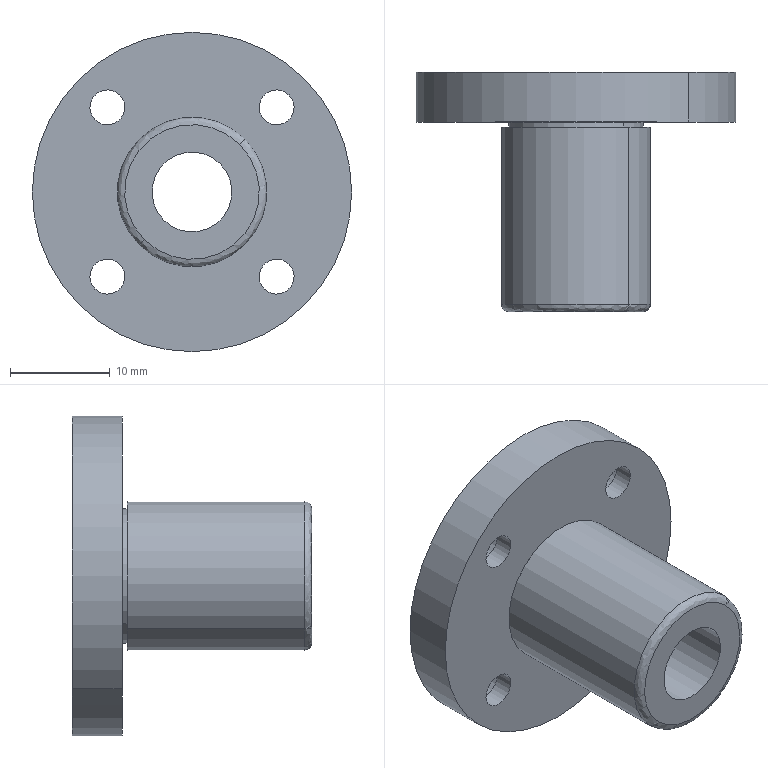Component | SolidWorks | LinearBearingLHFR8-1 | 1 solid | 34 faces | box 32 x 24 x 32 mm | volume 5726 mm3 | cylinder 24 | plane 7 | spline 3 | commonest cylinder face diameters 6 x8 3.5 x8 32 x2 8 x2 13.5 x2 15 x2
STEP:
#1=COLOUR_RGB('',0.7922,0.8196,0.9333);
#2=FILL_AREA_STYLE_COLOUR('',#1);
#3=FILL_AREA_STYLE('',(#2));
#4=SURFACE_STYLE_FILL_AREA(#3);
#5=SURFACE_SIDE_STYLE('',(#4));
#6=SURFACE_STYLE_USAGE(.BOTH.,#5);
#7=PRESENTATION_STYLE_ASSIGNMENT((#6));
#8=CARTESIAN_POINT('',(0.03812,2.123,-4.792));
#9=VERTEX_POINT('',#8);
#10=CARTESIAN_POINT('',(-0.3795,2.123,-5.209));
#11=VERTEX_POINT('',#10);
#12=CARTESIAN_POINT('',(-0.1707,2.123,-5.001));
#13=DIRECTION('',(0.,-1.,0.));
#14=DIRECTION('',(0.7071,0.,0.7071));
#15=AXIS2_PLACEMENT_3D('',#12,#13,#14);
#16=CIRCLE('',#15,0.2953);
#17=EDGE_CURVE('',#9,#11,#16,.T.);
#18=ORIENTED_EDGE('',*,*,#17,.T.);
#19=CARTESIAN_POINT('',(-0.3586,2.093,-5.188));
#20=VERTEX_POINT('',#19);
#21=CARTESIAN_POINT('',(-0.3586,2.123,-5.188));
#22=DIRECTION('',(-0.7071,0.,0.7071));
#23=DIRECTION('',(0.7071,0.,0.7071));
#24=AXIS2_PLACEMENT_3D('',#21,#22,#23);
#25=CIRCLE('',#24,0.02953);
#26=EDGE_CURVE('',#11,#20,#25,.T.);
#27=ORIENTED_EDGE('',*,*,#26,.T.);
#28=CARTESIAN_POINT('',(0.01724,2.093,-4.813));
#29=VERTEX_POINT('',#28);
#30=CARTESIAN_POINT('',(-0.1707,2.093,-5.001));
#31=DIRECTION('',(0.,-1.,0.));
#32=DIRECTION('',(0.7071,0.,0.7071));
#33=AXIS2_PLACEMENT_3D('',#30,#31,#32);
#34=CIRCLE('',#33,0.2657);
#35=EDGE_CURVE('',#29,#20,#34,.T.);
#36=ORIENTED_EDGE('',*,*,#35,.F.);
#37=CARTESIAN_POINT('',(0.01724,2.123,-4.813));
#38=DIRECTION('',(0.7071,0.,-0.7071));
#39=DIRECTION('',(-0.7071,0.,-0.7071));
#40=AXIS2_PLACEMENT_3D('',#37,#38,#39);
#41=CIRCLE('',#40,0.02953);
#42=EDGE_CURVE('',#9,#29,#41,.T.);
#43=ORIENTED_EDGE('',*,*,#42,.F.);
#44=EDGE_LOOP('',(#18,#27,#36,#43));
#45=FACE_OUTER_BOUND('',#44,.T.);
#46=CARTESIAN_POINT('',(-0.3795,2.123,-5.209));
#47=CARTESIAN_POINT('',(-0.7971,2.123,-4.792));
#48=CARTESIAN_POINT('',(-0.3795,2.123,-4.374));
#49=CARTESIAN_POINT('',(0.03812,2.123,-4.792));
#50=CARTESIAN_POINT('',(-0.3795,2.105,-5.209));
#51=CARTESIAN_POINT('',(-0.7971,2.105,-4.792));
#52=CARTESIAN_POINT('',(-0.3795,2.105,-4.374));
#53=CARTESIAN_POINT('',(0.03812,2.105,-4.792));
#54=CARTESIAN_POINT('',(-0.3708,2.093,-5.201));
#55=CARTESIAN_POINT('',(-0.7711,2.093,-4.8));
#56=CARTESIAN_POINT('',(-0.3708,2.093,-4.4));
#57=CARTESIAN_POINT('',(0.02947,2.093,-4.8));
#58=CARTESIAN_POINT('',(-0.3586,2.093,-5.188));
#59=CARTESIAN_POINT('',(-0.7344,2.093,-4.813));
#60=CARTESIAN_POINT('',(-0.3586,2.093,-4.437));
#61=CARTESIAN_POINT('',(0.01724,2.093,-4.813));
#62=(BOUNDED_SURFACE()B_SPLINE_SURFACE(3,3,((#46,#47,#48,#49),(#50,#51,#52,#53),(#54,#55,#56,#57),(#58,#59,#60,#61)),.UNSPECIFIED.,.F.,.F.,.T.)B_SPLINE_SURFACE_WITH_KNOTS((4,4),(4,4),(0.,1.),(0.,1.),.UNSPECIFIED.)GEOMETRIC_REPRESENTATION_ITEM()RATIONAL_B_SPLINE_SURFACE(((1.,0.3333,0.3333,1.),(0.8047,0.2682,0.2682,0.8047),(0.8047,0.2682,0.2682,0.8047),(1.,0.3333,0.3333,1.)))REPRESENTATION_ITEM('')SURFACE());
#63=ADVANCED_FACE('',(#45),#62,.T.);
#64=CARTESIAN_POINT('',(0.2747,2.841,-4.555));
#65=VERTEX_POINT('',#64);
#66=CARTESIAN_POINT('',(-0.6161,2.841,-5.446));
#67=VERTEX_POINT('',#66);
#68=CARTESIAN_POINT('',(-0.1707,2.841,-5.001));
#69=DIRECTION('',(0.,1.,0.));
#70=DIRECTION('',(0.7071,0.,0.7071));
#71=AXIS2_PLACEMENT_3D('',#68,#69,#70);
#72=CIRCLE('',#71,0.6299);
#73=EDGE_CURVE('',#65,#67,#72,.T.);
#74=ORIENTED_EDGE('',*,*,#73,.T.);
#75=CARTESIAN_POINT('',(-0.6161,3.038,-5.446));
#76=VERTEX_POINT('',#75);
#77=CARTESIAN_POINT('',(-0.6161,3.038,-5.446));
#78=DIRECTION('',(0.,1.,0.));
#79=VECTOR('',#78,39.37);
#80=LINE('',#77,#79);
#81=EDGE_CURVE('',#67,#76,#80,.T.);
#82=ORIENTED_EDGE('',*,*,#81,.T.);
#83=CARTESIAN_POINT('',(0.2747,3.038,-4.555));
#84=VERTEX_POINT('',#83);
#85=CARTESIAN_POINT('',(-0.1707,3.038,-5.001));
#86=DIRECTION('',(0.,-1.,0.));
#87=DIRECTION('',(0.7071,0.,0.7071));
#88=AXIS2_PLACEMENT_3D('',#85,#86,#87);
#89=CIRCLE('',#88,0.6299);
#90=EDGE_CURVE('',#76,#84,#89,.T.);
#91=ORIENTED_EDGE('',*,*,#90,.T.);
#92=CARTESIAN_POINT('',(0.2747,3.038,-4.555));
#93=DIRECTION('',(0.,1.,0.));
#94=VECTOR('',#93,39.37);
#95=LINE('',#92,#94);
#96=EDGE_CURVE('',#65,#84,#95,.T.);
#97=ORIENTED_EDGE('',*,*,#96,.F.);
#98=EDGE_LOOP('',(#74,#82,#91,#97));
#99=FACE_OUTER_BOUND('',#98,.T.);
#100=CARTESIAN_POINT('',(-0.1707,3.038,-5.001));
#101=DIRECTION('',(0.,1.,0.));
#102=DIRECTION('',(0.7071,0.,0.7071));
#103=AXIS2_PLACEMENT_3D('',#100,#101,#102);
#104=CYLINDRICAL_SURFACE('',#103,0.6299);
#105=ADVANCED_FACE('',(#99),#104,.T.);
#106=CARTESIAN_POINT('',(-0.05932,2.093,-4.889));
#107=VERTEX_POINT('',#106);
#108=CARTESIAN_POINT('',(-0.282,2.093,-5.112));
#109=VERTEX_POINT('',#108);
#110=CARTESIAN_POINT('',(-0.1707,2.093,-5.001));
#111=DIRECTION('',(0.,-1.,0.));
#112=DIRECTION('',(0.7071,0.,0.7071));
#113=AXIS2_PLACEMENT_3D('',#110,#111,#112);
#114=CIRCLE('',#113,0.1575);
#115=EDGE_CURVE('',#107,#109,#114,.T.);
#116=ORIENTED_EDGE('',*,*,#115,.T.);
#117=CARTESIAN_POINT('',(-0.282,3.038,-5.112));
#118=VERTEX_POINT('',#117);
#119=CARTESIAN_POINT('',(-0.282,2.093,-5.112));
#120=DIRECTION('',(0.,1.,0.));
#121=VECTOR('',#120,39.37);
#122=LINE('',#119,#121);
#123=EDGE_CURVE('',#109,#118,#122,.T.);
#124=ORIENTED_EDGE('',*,*,#123,.T.);
#125=CARTESIAN_POINT('',(-0.05932,3.038,-4.889));
#126=VERTEX_POINT('',#125);
#127=CARTESIAN_POINT('',(-0.1707,3.038,-5.001));
#128=DIRECTION('',(0.,-1.,0.));
#129=DIRECTION('',(0.7071,0.,0.7071));
#130=AXIS2_PLACEMENT_3D('',#127,#128,#129);
#131=CIRCLE('',#130,0.1575);
#132=EDGE_CURVE('',#126,#118,#131,.T.);
#133=ORIENTED_EDGE('',*,*,#132,.F.);
#134=CARTESIAN_POINT('',(-0.05932,2.093,-4.889));
#135=DIRECTION('',(0.,1.,0.));
#136=VECTOR('',#135,39.37);
#137=LINE('',#134,#136);
#138=EDGE_CURVE('',#107,#126,#137,.T.);
#139=ORIENTED_EDGE('',*,*,#138,.F.);
#140=EDGE_LOOP('',(#116,#124,#133,#139));
#141=FACE_OUTER_BOUND('',#140,.T.);
#142=CARTESIAN_POINT('',(-0.1707,2.093,-5.001));
#143=DIRECTION('',(0.,1.,0.));
#144=DIRECTION('',(0.7071,0.,0.7071));
#145=AXIS2_PLACEMENT_3D('',#142,#143,#144);
#146=CYLINDRICAL_SURFACE('',#145,0.1575);
#147=ADVANCED_FACE('',(#141),#146,.F.);
#148=CARTESIAN_POINT('',(0.2469,2.916,-5.251));
#149=VERTEX_POINT('',#148);
#150=CARTESIAN_POINT('',(0.07987,2.916,-5.418));
#151=VERTEX_POINT('',#150);
#152=CARTESIAN_POINT('',(0.1634,2.916,-5.335));
#153=DIRECTION('',(0.,-1.,0.));
#154=DIRECTION('',(0.7071,0.,0.7071));
#155=AXIS2_PLACEMENT_3D('',#152,#153,#154);
#156=CIRCLE('',#155,0.1181);
#157=EDGE_CURVE('',#149,#151,#156,.T.);
#158=ORIENTED_EDGE('',*,*,#157,.T.);
#159=CARTESIAN_POINT('',(0.07987,3.038,-5.418));
#160=VERTEX_POINT('',#159);
#161=CARTESIAN_POINT('',(0.07987,2.916,-5.418));
#162=DIRECTION('',(0.,1.,0.));
#163=VECTOR('',#162,39.37);
#164=LINE('',#161,#163);
#165=EDGE_CURVE('',#151,#160,#164,.T.);
#166=ORIENTED_EDGE('',*,*,#165,.T.);
#167=CARTESIAN_POINT('',(0.2469,3.038,-5.251));
#168=VERTEX_POINT('',#167);
#169=CARTESIAN_POINT('',(0.1634,3.038,-5.335));
#170=DIRECTION('',(0.,-1.,0.));
#171=DIRECTION('',(0.7071,0.,0.7071));
#172=AXIS2_PLACEMENT_3D('',#169,#170,#171);
#173=CIRCLE('',#172,0.1181);
#174=EDGE_CURVE('',#168,#160,#173,.T.);
#175=ORIENTED_EDGE('',*,*,#174,.F.);
#176=CARTESIAN_POINT('',(0.2469,2.916,-5.251));
#177=DIRECTION('',(0.,1.,0.));
#178=VECTOR('',#177,39.37);
#179=LINE('',#176,#178);
#180=EDGE_CURVE('',#149,#168,#179,.T.);
#181=ORIENTED_EDGE('',*,*,#180,.F.);
#182=EDGE_LOOP('',(#158,#166,#175,#181));
#183=FACE_OUTER_BOUND('',#182,.T.);
#184=CARTESIAN_POINT('',(0.1634,2.916,-5.335));
#185=DIRECTION('',(0.,1.,0.));
#186=DIRECTION('',(0.7071,0.,0.7071));
#187=AXIS2_PLACEMENT_3D('',#184,#185,#186);
#188=CYLINDRICAL_SURFACE('',#187,0.1181);
#189=ADVANCED_FACE('',(#183),#188,.F.);
#190=CARTESIAN_POINT('',(-0.4212,2.916,-5.251));
#191=VERTEX_POINT('',#190);
#192=CARTESIAN_POINT('',(-0.5883,2.916,-5.418));
#193=VERTEX_POINT('',#192);
#194=CARTESIAN_POINT('',(-0.5047,2.916,-5.335));
#195=DIRECTION('',(0.,-1.,0.));
#196=DIRECTION('',(0.7071,0.,0.7071));
#197=AXIS2_PLACEMENT_3D('',#194,#195,#196);
#198=CIRCLE('',#197,0.1181);
#199=EDGE_CURVE('',#191,#193,#198,.T.);
#200=ORIENTED_EDGE('',*,*,#199,.T.);
#201=CARTESIAN_POINT('',(-0.5883,3.038,-5.418));
#202=VERTEX_POINT('',#201);
#203=CARTESIAN_POINT('',(-0.5883,2.916,-5.418));
#204=DIRECTION('',(0.,1.,0.));
#205=VECTOR('',#204,39.37);
#206=LINE('',#203,#205);
#207=EDGE_CURVE('',#193,#202,#206,.T.);
#208=ORIENTED_EDGE('',*,*,#207,.T.);
#209=CARTESIAN_POINT('',(-0.4212,3.038,-5.251));
#210=VERTEX_POINT('',#209);
#211=CARTESIAN_POINT('',(-0.5047,3.038,-5.335));
#212=DIRECTION('',(0.,-1.,0.));
#213=DIRECTION('',(0.7071,0.,0.7071));
#214=AXIS2_PLACEMENT_3D('',#211,#212,#213);
#215=CIRCLE('',#214,0.1181);
#216=EDGE_CURVE('',#210,#202,#215,.T.);
#217=ORIENTED_EDGE('',*,*,#216,.F.);
#218=CARTESIAN_POINT('',(-0.4212,2.916,-5.251));
#219=DIRECTION('',(0.,1.,0.));
#220=VECTOR('',#219,39.37);
#221=LINE('',#218,#220);
#222=EDGE_CURVE('',#191,#210,#221,.T.);
#223=ORIENTED_EDGE('',*,*,#222,.F.);
#224=EDGE_LOOP('',(#200,#208,#217,#223));
#225=FACE_OUTER_BOUND('',#224,.T.);
#226=CARTESIAN_POINT('',(-0.5047,2.916,-5.335));
#227=DIRECTION('',(0.,1.,0.));
#228=DIRECTION('',(0.7071,0.,0.7071));
#229=AXIS2_PLACEMENT_3D('',#226,#227,#228);
#230=CYLINDRICAL_SURFACE('',#229,0.1181);
#231=ADVANCED_FACE('',(#225),#230,.F.);
#232=CARTESIAN_POINT('',(-0.4212,2.916,-4.583));
#233=VERTEX_POINT('',#232);
#234=CARTESIAN_POINT('',(-0.5883,2.916,-4.75));
#235=VERTEX_POINT('',#234);
#236=CARTESIAN_POINT('',(-0.5047,2.916,-4.667));
#237=DIRECTION('',(0.,-1.,0.));
#238=DIRECTION('',(0.7071,0.,0.7071));
#239=AXIS2_PLACEMENT_3D('',#236,#237,#238);
#240=CIRCLE('',#239,0.1181);
#241=EDGE_CURVE('',#233,#235,#240,.T.);
#242=ORIENTED_EDGE('',*,*,#241,.T.);
#243=CARTESIAN_POINT('',(-0.5883,3.038,-4.75));
#244=VERTEX_POINT('',#243);
#245=CARTESIAN_POINT('',(-0.5883,2.916,-4.75));
#246=DIRECTION('',(0.,1.,0.));
#247=VECTOR('',#246,39.37);
#248=LINE('',#245,#247);
#249=EDGE_CURVE('',#235,#244,#248,.T.);
#250=ORIENTED_EDGE('',*,*,#249,.T.);
#251=CARTESIAN_POINT('',(-0.4212,3.038,-4.583));
#252=VERTEX_POINT('',#251);
#253=CARTESIAN_POINT('',(-0.5047,3.038,-4.667));
#254=DIRECTION('',(0.,-1.,0.));
#255=DIRECTION('',(0.7071,0.,0.7071));
#256=AXIS2_PLACEMENT_3D('',#253,#254,#255);
#257=CIRCLE('',#256,0.1181);
#258=EDGE_CURVE('',#252,#244,#257,.T.);
#259=ORIENTED_EDGE('',*,*,#258,.F.);
#260=CARTESIAN_POINT('',(-0.4212,2.916,-4.583));
#261=DIRECTION('',(0.,1.,0.));
#262=VECTOR('',#261,39.37);
#263=LINE('',#260,#262);
#264=EDGE_CURVE('',#233,#252,#263,.T.);
#265=ORIENTED_EDGE('',*,*,#264,.F.);
#266=EDGE_LOOP('',(#242,#250,#259,#265));
#267=FACE_OUTER_BOUND('',#266,.T.);
#268=CARTESIAN_POINT('',(-0.5047,2.916,-4.667));
#269=DIRECTION('',(0.,1.,0.));
#270=DIRECTION('',(0.7071,0.,0.7071));
#271=AXIS2_PLACEMENT_3D('',#268,#269,#270);
#272=CYLINDRICAL_SURFACE('',#271,0.1181);
#273=ADVANCED_FACE('',(#267),#272,.F.);
#274=CARTESIAN_POINT('',(0.2469,2.916,-4.583));
#275=VERTEX_POINT('',#274);
#276=CARTESIAN_POINT('',(0.07987,2.916,-4.75));
#277=VERTEX_POINT('',#276);
#278=CARTESIAN_POINT('',(0.1634,2.916,-4.667));
#279=DIRECTION('',(0.,-1.,0.));
#280=DIRECTION('',(0.7071,0.,0.7071));
#281=AXIS2_PLACEMENT_3D('',#278,#279,#280);
#282=CIRCLE('',#281,0.1181);
#283=EDGE_CURVE('',#275,#277,#282,.T.);
#284=ORIENTED_EDGE('',*,*,#283,.T.);
#285=CARTESIAN_POINT('',(0.07987,3.038,-4.75));
#286=VERTEX_POINT('',#285);
#287=CARTESIAN_POINT('',(0.07987,2.916,-4.75));
#288=DIRECTION('',(0.,1.,0.));
#289=VECTOR('',#288,39.37);
#290=LINE('',#287,#289);
#291=EDGE_CURVE('',#277,#286,#290,.T.);
#292=ORIENTED_EDGE('',*,*,#291,.T.);
#293=CARTESIAN_POINT('',(0.2469,3.038,-4.583));
#294=VERTEX_POINT('',#293);
#295=CARTESIAN_POINT('',(0.1634,3.038,-4.667));
#296=DIRECTION('',(0.,-1.,0.));
#297=DIRECTION('',(0.7071,0.,0.7071));
#298=AXIS2_PLACEMENT_3D('',#295,#296,#297);
#299=CIRCLE('',#298,0.1181);
#300=EDGE_CURVE('',#294,#286,#299,.T.);
#301=ORIENTED_EDGE('',*,*,#300,.F.);
#302=CARTESIAN_POINT('',(0.2469,2.916,-4.583));
#303=DIRECTION('',(0.,1.,0.));
#304=VECTOR('',#303,39.37);
#305=LINE('',#302,#304);
#306=EDGE_CURVE('',#275,#294,#305,.T.);
#307=ORIENTED_EDGE('',*,*,#306,.F.);
#308=EDGE_LOOP('',(#284,#292,#301,#307));
#309=FACE_OUTER_BOUND('',#308,.T.);
#310=CARTESIAN_POINT('',(0.1634,2.916,-4.667));
#311=DIRECTION('',(0.,1.,0.));
#312=DIRECTION('',(0.7071,0.,0.7071));
#313=AXIS2_PLACEMENT_3D('',#310,#311,#312);
#314=CYLINDRICAL_SURFACE('',#313,0.1181);
#315=ADVANCED_FACE('',(#309),#314,.F.);
#316=CARTESIAN_POINT('',(0.01724,2.822,-4.813));
#317=VERTEX_POINT('',#316);
#318=CARTESIAN_POINT('',(-0.3586,2.822,-5.188));
#319=VERTEX_POINT('',#318);
#320=CARTESIAN_POINT('',(-0.1707,2.822,-5.001));
#321=DIRECTION('',(0.,1.,0.));
#322=DIRECTION('',(0.7071,0.,0.7071));
#323=AXIS2_PLACEMENT_3D('',#320,#321,#322);
#324=CIRCLE('',#323,0.2657);
#325=EDGE_CURVE('',#317,#319,#324,.T.);
#326=ORIENTED_EDGE('',*,*,#325,.T.);
#327=CARTESIAN_POINT('',(-0.3586,2.841,-5.188));
#328=VERTEX_POINT('',#327);
#329=CARTESIAN_POINT('',(-0.3586,2.841,-5.188));
#330=DIRECTION('',(0.,1.,0.));
#331=VECTOR('',#330,39.37);
#332=LINE('',#329,#331);
#333=EDGE_CURVE('',#319,#328,#332,.T.);
#334=ORIENTED_EDGE('',*,*,#333,.T.);
#335=CARTESIAN_POINT('',(0.01724,2.841,-4.813));
#336=VERTEX_POINT('',#335);
#337=CARTESIAN_POINT('',(-0.1707,2.841,-5.001));
#338=DIRECTION('',(0.,1.,0.));
#339=DIRECTION('',(0.7071,0.,0.7071));
#340=AXIS2_PLACEMENT_3D('',#337,#338,#339);
#341=CIRCLE('',#340,0.2657);
#342=EDGE_CURVE('',#336,#328,#341,.T.);
#343=ORIENTED_EDGE('',*,*,#342,.F.);
#344=CARTESIAN_POINT('',(0.01724,2.841,-4.813));
#345=DIRECTION('',(0.,1.,0.));
#346=VECTOR('',#345,39.37);
#347=LINE('',#344,#346);
#348=EDGE_CURVE('',#317,#336,#347,.T.);
#349=ORIENTED_EDGE('',*,*,#348,.F.);
#350=EDGE_LOOP('',(#326,#334,#343,#349));
#351=FACE_OUTER_BOUND('',#350,.T.);
#352=CARTESIAN_POINT('',(-0.1707,2.841,-5.001));
#353=DIRECTION('',(0.,1.,0.));
#354=DIRECTION('',(0.7071,0.,0.7071));
#355=AXIS2_PLACEMENT_3D('',#352,#353,#354);
#356=CYLINDRICAL_SURFACE('',#355,0.2657);
#357=ADVANCED_FACE('',(#351),#356,.T.);
#358=CARTESIAN_POINT('',(0.1147,2.841,-5.383));
#359=VERTEX_POINT('',#358);
#360=CARTESIAN_POINT('',(0.2121,2.841,-5.286));
#361=VERTEX_POINT('',#360);
#362=CARTESIAN_POINT('',(0.1634,2.841,-5.335));
#363=DIRECTION('',(0.,1.,0.));
#364=DIRECTION('',(0.7071,0.,0.7071));
#365=AXIS2_PLACEMENT_3D('',#362,#363,#364);
#366=CIRCLE('',#365,0.0689);
#367=EDGE_CURVE('',#359,#361,#366,.T.);
#368=ORIENTED_EDGE('',*,*,#367,.F.);
#369=CARTESIAN_POINT('',(0.1147,2.916,-5.383));
#370=VERTEX_POINT('',#369);
#371=CARTESIAN_POINT('',(0.1147,2.841,-5.383));
#372=DIRECTION('',(0.,1.,0.));
#373=VECTOR('',#372,39.37);
#374=LINE('',#371,#373);
#375=EDGE_CURVE('',#359,#370,#374,.T.);
#376=ORIENTED_EDGE('',*,*,#375,.T.);
#377=CARTESIAN_POINT('',(0.2121,2.916,-5.286));
#378=VERTEX_POINT('',#377);
#379=CARTESIAN_POINT('',(0.1634,2.916,-5.335));
#380=DIRECTION('',(0.,1.,0.));
#381=DIRECTION('',(0.7071,0.,0.7071));
#382=AXIS2_PLACEMENT_3D('',#379,#380,#381);
#383=CIRCLE('',#382,0.0689);
#384=EDGE_CURVE('',#370,#378,#383,.T.);
#385=ORIENTED_EDGE('',*,*,#384,.T.);
#386=CARTESIAN_POINT('',(0.2121,2.841,-5.286));
#387=DIRECTION('',(0.,1.,0.));
#388=VECTOR('',#387,39.37);
#389=LINE('',#386,#388);
#390=EDGE_CURVE('',#361,#378,#389,.T.);
#391=ORIENTED_EDGE('',*,*,#390,.F.);
#392=EDGE_LOOP('',(#368,#376,#385,#391));
#393=FACE_OUTER_BOUND('',#392,.T.);
#394=CARTESIAN_POINT('',(0.1634,2.841,-5.335));
#395=DIRECTION('',(0.,1.,0.));
#396=DIRECTION('',(0.7071,0.,0.7071));
#397=AXIS2_PLACEMENT_3D('',#394,#395,#396);
#398=CYLINDRICAL_SURFACE('',#397,0.0689);
#399=ADVANCED_FACE('',(#393),#398,.F.);
#400=CARTESIAN_POINT('',(-0.5535,2.841,-5.383));
#401=VERTEX_POINT('',#400);
#402=CARTESIAN_POINT('',(-0.456,2.841,-5.286));
#403=VERTEX_POINT('',#402);
#404=CARTESIAN_POINT('',(-0.5047,2.841,-5.335));
#405=DIRECTION('',(0.,1.,0.));
#406=DIRECTION('',(0.7071,0.,0.7071));
#407=AXIS2_PLACEMENT_3D('',#404,#405,#406);
#408=CIRCLE('',#407,0.0689);
#409=EDGE_CURVE('',#401,#403,#408,.T.);
#410=ORIENTED_EDGE('',*,*,#409,.F.);
#411=CARTESIAN_POINT('',(-0.5535,2.916,-5.383));
#412=VERTEX_POINT('',#411);
#413=CARTESIAN_POINT('',(-0.5535,2.841,-5.383));
#414=DIRECTION('',(0.,1.,0.));
#415=VECTOR('',#414,39.37);
#416=LINE('',#413,#415);
#417=EDGE_CURVE('',#401,#412,#416,.T.);
#418=ORIENTED_EDGE('',*,*,#417,.T.);
#419=CARTESIAN_POINT('',(-0.456,2.916,-5.286));
#420=VERTEX_POINT('',#419);
#421=CARTESIAN_POINT('',(-0.5047,2.916,-5.335));
#422=DIRECTION('',(0.,1.,0.));
#423=DIRECTION('',(0.7071,0.,0.7071));
#424=AXIS2_PLACEMENT_3D('',#421,#422,#423);
#425=CIRCLE('',#424,0.0689);
#426=EDGE_CURVE('',#412,#420,#425,.T.);
#427=ORIENTED_EDGE('',*,*,#426,.T.);
#428=CARTESIAN_POINT('',(-0.456,2.841,-5.286));
#429=DIRECTION('',(0.,1.,0.));
#430=VECTOR('',#429,39.37);
#431=LINE('',#428,#430);
#432=EDGE_CURVE('',#403,#420,#431,.T.);
#433=ORIENTED_EDGE('',*,*,#432,.F.);
#434=EDGE_LOOP('',(#410,#418,#427,#433));
#435=FACE_OUTER_BOUND('',#434,.T.);
#436=CARTESIAN_POINT('',(-0.5047,2.841,-5.335));
#437=DIRECTION('',(0.,1.,0.));
#438=DIRECTION('',(0.7071,0.,0.7071));
#439=AXIS2_PLACEMENT_3D('',#436,#437,#438);
#440=CYLINDRICAL_SURFACE('',#439,0.0689);
#441=ADVANCED_FACE('',(#435),#440,.F.);
#442=CARTESIAN_POINT('',(-0.5535,2.841,-4.715));
#443=VERTEX_POINT('',#442);
#444=CARTESIAN_POINT('',(-0.456,2.841,-4.618));
#445=VERTEX_POINT('',#444);
#446=CARTESIAN_POINT('',(-0.5047,2.841,-4.667));
#447=DIRECTION('',(0.,1.,0.));
#448=DIRECTION('',(0.7071,0.,0.7071));
#449=AXIS2_PLACEMENT_3D('',#446,#447,#448);
#450=CIRCLE('',#449,0.0689);
#451=EDGE_CURVE('',#443,#445,#450,.T.);
#452=ORIENTED_EDGE('',*,*,#451,.F.);
#453=CARTESIAN_POINT('',(-0.5535,2.916,-4.715));
#454=VERTEX_POINT('',#453);
#455=CARTESIAN_POINT('',(-0.5535,2.841,-4.715));
#456=DIRECTION('',(0.,1.,0.));
#457=VECTOR('',#456,39.37);
#458=LINE('',#455,#457);
#459=EDGE_CURVE('',#443,#454,#458,.T.);
#460=ORIENTED_EDGE('',*,*,#459,.T.);
#461=CARTESIAN_POINT('',(-0.456,2.916,-4.618));
#462=VERTEX_POINT('',#461);
#463=CARTESIAN_POINT('',(-0.5047,2.916,-4.667));
#464=DIRECTION('',(0.,1.,0.));
#465=DIRECTION('',(0.7071,0.,0.7071));
#466=AXIS2_PLACEMENT_3D('',#463,#464,#465);
#467=CIRCLE('',#466,0.0689);
#468=EDGE_CURVE('',#454,#462,#467,.T.);
#469=ORIENTED_EDGE('',*,*,#468,.T.);
#470=CARTESIAN_POINT('',(-0.456,2.841,-4.618));
#471=DIRECTION('',(0.,1.,0.));
#472=VECTOR('',#471,39.37);
#473=LINE('',#470,#472);
#474=EDGE_CURVE('',#445,#462,#473,.T.);
#475=ORIENTED_EDGE('',*,*,#474,.F.);
#476=EDGE_LOOP('',(#452,#460,#469,#475));
#477=FACE_OUTER_BOUND('',#476,.T.);
#478=CARTESIAN_POINT('',(-0.5047,2.841,-4.667));
#479=DIRECTION('',(0.,1.,0.));
#480=DIRECTION('',(0.7071,0.,0.7071));
#481=AXIS2_PLACEMENT_3D('',#478,#479,#480);
#482=CYLINDRICAL_SURFACE('',#481,0.0689);
#483=ADVANCED_FACE('',(#477),#482,.F.);
#484=CARTESIAN_POINT('',(0.1147,2.841,-4.715));
#485=VERTEX_POINT('',#484);
#486=CARTESIAN_POINT('',(0.2121,2.841,-4.618));
#487=VERTEX_POINT('',#486);
#488=CARTESIAN_POINT('',(0.1634,2.841,-4.667));
#489=DIRECTION('',(0.,1.,0.));
#490=DIRECTION('',(0.7071,0.,0.7071));
#491=AXIS2_PLACEMENT_3D('',#488,#489,#490);
#492=CIRCLE('',#491,0.0689);
#493=EDGE_CURVE('',#485,#487,#492,.T.);
#494=ORIENTED_EDGE('',*,*,#493,.F.);
#495=CARTESIAN_POINT('',(0.1147,2.916,-4.715));
#496=VERTEX_POINT('',#495);
#497=CARTESIAN_POINT('',(0.1147,2.841,-4.715));
#498=DIRECTION('',(0.,1.,0.));
#499=VECTOR('',#498,39.37);
#500=LINE('',#497,#499);
#501=EDGE_CURVE('',#485,#496,#500,.T.);
#502=ORIENTED_EDGE('',*,*,#501,.T.);
#503=CARTESIAN_POINT('',(0.2121,2.916,-4.618));
#504=VERTEX_POINT('',#503);
#505=CARTESIAN_POINT('',(0.1634,2.916,-4.667));
#506=DIRECTION('',(0.,1.,0.));
#507=DIRECTION('',(0.7071,0.,0.7071));
#508=AXIS2_PLACEMENT_3D('',#505,#506,#507);
#509=CIRCLE('',#508,0.0689);
#510=EDGE_CURVE('',#496,#504,#509,.T.);
#511=ORIENTED_EDGE('',*,*,#510,.T.);
#512=CARTESIAN_POINT('',(0.2121,2.841,-4.618));
#513=DIRECTION('',(0.,1.,0.));
#514=VECTOR('',#513,39.37);
#515=LINE('',#512,#514);
#516=EDGE_CURVE('',#487,#504,#515,.T.);
#517=ORIENTED_EDGE('',*,*,#516,.F.);
#518=EDGE_LOOP('',(#494,#502,#511,#517));
#519=FACE_OUTER_BOUND('',#518,.T.);
#520=CARTESIAN_POINT('',(0.1634,2.841,-4.667));
#521=DIRECTION('',(0.,1.,0.));
#522=DIRECTION('',(0.7071,0.,0.7071));
#523=AXIS2_PLACEMENT_3D('',#520,#521,#522);
#524=CYLINDRICAL_SURFACE('',#523,0.0689);
#525=ADVANCED_FACE('',(#519),#524,.F.);
#526=CARTESIAN_POINT('',(-0.1707,2.123,-5.001));
#527=DIRECTION('',(0.,-1.,0.));
#528=DIRECTION('',(0.7071,0.,0.7071));
#529=AXIS2_PLACEMENT_3D('',#526,#527,#528);
#530=CIRCLE('',#529,0.2953);
#531=EDGE_CURVE('',#11,#9,#530,.T.);
#532=ORIENTED_EDGE('',*,*,#531,.F.);
#533=CARTESIAN_POINT('',(-0.3795,2.822,-5.209));
#534=VERTEX_POINT('',#533);
#535=CARTESIAN_POINT('',(-0.3795,2.822,-5.209));
#536=DIRECTION('',(0.,1.,0.));
#537=VECTOR('',#536,39.37);
#538=LINE('',#535,#537);
#539=EDGE_CURVE('',#11,#534,#538,.T.);
#540=ORIENTED_EDGE('',*,*,#539,.T.);
#541=CARTESIAN_POINT('',(0.03812,2.822,-4.792));
#542=VERTEX_POINT('',#541);
#543=CARTESIAN_POINT('',(-0.1707,2.822,-5.001));
#544=DIRECTION('',(0.,1.,0.));
#545=DIRECTION('',(0.7071,0.,0.7071));
#546=AXIS2_PLACEMENT_3D('',#543,#544,#545);
#547=CIRCLE('',#546,0.2953);
#548=EDGE_CURVE('',#542,#534,#547,.T.);
#549=ORIENTED_EDGE('',*,*,#548,.F.);
#550=CARTESIAN_POINT('',(0.03812,2.822,-4.792));
#551=DIRECTION('',(0.,1.,0.));
#552=VECTOR('',#551,39.37);
#553=LINE('',#550,#552);
#554=EDGE_CURVE('',#9,#542,#553,.T.);
#555=ORIENTED_EDGE('',*,*,#554,.F.);
#556=EDGE_LOOP('',(#532,#540,#549,#555));
#557=FACE_OUTER_BOUND('',#556,.T.);
#558=CARTESIAN_POINT('',(-0.1707,2.822,-5.001));
#559=DIRECTION('',(0.,1.,0.));
#560=DIRECTION('',(0.7071,0.,0.7071));
#561=AXIS2_PLACEMENT_3D('',#558,#559,#560);
#562=CYLINDRICAL_SURFACE('',#561,0.2953);
#563=ADVANCED_FACE('',(#557),#562,.T.);
#564=ORIENTED_EDGE('',*,*,#81,.F.);
#565=CARTESIAN_POINT('',(-0.1707,2.841,-5.001));
#566=DIRECTION('',(0.,1.,0.));
#567=DIRECTION('',(0.7071,0.,0.7071));
#568=AXIS2_PLACEMENT_3D('',#565,#566,#567);
#569=CIRCLE('',#568,0.6299);
#570=EDGE_CURVE('',#67,#65,#569,.T.);
#571=ORIENTED_EDGE('',*,*,#570,.T.);
#572=ORIENTED_EDGE('',*,*,#96,.T.);
#573=CARTESIAN_POINT('',(-0.1707,3.038,-5.001));
#574=DIRECTION('',(0.,-1.,0.));
#575=DIRECTION('',(0.7071,0.,0.7071));
#576=AXIS2_PLACEMENT_3D('',#573,#574,#575);
#577=CIRCLE('',#576,0.6299);
#578=EDGE_CURVE('',#84,#76,#577,.T.);
#579=ORIENTED_EDGE('',*,*,#578,.T.);
#580=EDGE_LOOP('',(#564,#571,#572,#579));
#581=FACE_OUTER_BOUND('',#580,.T.);
#582=CARTESIAN_POINT('',(-0.1707,3.038,-5.001));
#583=DIRECTION('',(0.,1.,0.));
#584=DIRECTION('',(0.7071,0.,0.7071));
#585=AXIS2_PLACEMENT_3D('',#582,#583,#584);
#586=CYLINDRICAL_SURFACE('',#585,0.6299);
#587=ADVANCED_FACE('',(#581),#586,.T.);
#588=ORIENTED_EDGE('',*,*,#132,.T.);
#589=CARTESIAN_POINT('',(-0.1707,3.038,-5.001));
#590=DIRECTION('',(0.,-1.,0.));
#591=DIRECTION('',(0.7071,0.,0.7071));
#592=AXIS2_PLACEMENT_3D('',#589,#590,#591);
#593=CIRCLE('',#592,0.1575);
#594=EDGE_CURVE('',#118,#126,#593,.T.);
#595=ORIENTED_EDGE('',*,*,#594,.T.);
#596=EDGE_LOOP('',(#588,#595));
#597=FACE_BOUND('',#596,.T.);
#598=ORIENTED_EDGE('',*,*,#174,.T.);
#599=CARTESIAN_POINT('',(0.1634,3.038,-5.335));
#600=DIRECTION('',(0.,-1.,0.));
#601=DIRECTION('',(0.7071,0.,0.7071));
#602=AXIS2_PLACEMENT_3D('',#599,#600,#601);
#603=CIRCLE('',#602,0.1181);
#604=EDGE_CURVE('',#160,#168,#603,.T.);
#605=ORIENTED_EDGE('',*,*,#604,.T.);
#606=EDGE_LOOP('',(#598,#605));
#607=FACE_BOUND('',#606,.T.);
#608=ORIENTED_EDGE('',*,*,#216,.T.);
#609=CARTESIAN_POINT('',(-0.5047,3.038,-5.335));
#610=DIRECTION('',(0.,-1.,0.));
#611=DIRECTION('',(0.7071,0.,0.7071));
#612=AXIS2_PLACEMENT_3D('',#609,#610,#611);
#613=CIRCLE('',#612,0.1181);
#614=EDGE_CURVE('',#202,#210,#613,.T.);
#615=ORIENTED_EDGE('',*,*,#614,.T.);
#616=EDGE_LOOP('',(#608,#615));
#617=FACE_BOUND('',#616,.T.);
#618=ORIENTED_EDGE('',*,*,#258,.T.);
#619=CARTESIAN_POINT('',(-0.5047,3.038,-4.667));
#620=DIRECTION('',(0.,-1.,0.));
#621=DIRECTION('',(0.7071,0.,0.7071));
#622=AXIS2_PLACEMENT_3D('',#619,#620,#621);
#623=CIRCLE('',#622,0.1181);
#624=EDGE_CURVE('',#244,#252,#623,.T.);
#625=ORIENTED_EDGE('',*,*,#624,.T.);
#626=EDGE_LOOP('',(#618,#625));
#627=FACE_BOUND('',#626,.T.);
#628=ORIENTED_EDGE('',*,*,#300,.T.);
#629=CARTESIAN_POINT('',(0.1634,3.038,-4.667));
#630=DIRECTION('',(0.,-1.,0.));
#631=DIRECTION('',(0.7071,0.,0.7071));
#632=AXIS2_PLACEMENT_3D('',#629,#630,#631);
#633=CIRCLE('',#632,0.1181);
#634=EDGE_CURVE('',#286,#294,#633,.T.);
#635=ORIENTED_EDGE('',*,*,#634,.T.);
#636=EDGE_LOOP('',(#628,#635));
#637=FACE_BOUND('',#636,.T.);
#638=ORIENTED_EDGE('',*,*,#578,.F.);
#639=ORIENTED_EDGE('',*,*,#90,.F.);
#640=EDGE_LOOP('',(#638,#639));
#641=FACE_OUTER_BOUND('',#640,.T.);
#642=CARTESIAN_POINT('',(-0.1653,3.038,-4.104));
#643=DIRECTION('',(0.,1.,0.));
#644=DIRECTION('',(0.7071,0.,-0.7071));
#645=AXIS2_PLACEMENT_3D('',#642,#643,#644);
#646=PLANE('',#645);
#647=ADVANCED_FACE('',(#597,#607,#617,#627,#637,#641),#646,.T.);
#648=ORIENTED_EDGE('',*,*,#342,.T.);
#649=CARTESIAN_POINT('',(-0.1707,2.841,-5.001));
#650=DIRECTION('',(0.,1.,0.));
#651=DIRECTION('',(0.7071,0.,0.7071));
#652=AXIS2_PLACEMENT_3D('',#649,#650,#651);
#653=CIRCLE('',#652,0.2657);
#654=EDGE_CURVE('',#328,#336,#653,.T.);
#655=ORIENTED_EDGE('',*,*,#654,.T.);
#656=EDGE_LOOP('',(#648,#655));
#657=FACE_BOUND('',#656,.T.);
#658=CARTESIAN_POINT('',(0.1634,2.841,-5.335));
#659=DIRECTION('',(0.,1.,0.));
#660=DIRECTION('',(0.7071,0.,0.7071));
#661=AXIS2_PLACEMENT_3D('',#658,#659,#660);
#662=CIRCLE('',#661,0.0689);
#663=EDGE_CURVE('',#361,#359,#662,.T.);
#664=ORIENTED_EDGE('',*,*,#663,.T.);
#665=ORIENTED_EDGE('',*,*,#367,.T.);
#666=EDGE_LOOP('',(#664,#665));
#667=FACE_BOUND('',#666,.T.);
#668=CARTESIAN_POINT('',(-0.5047,2.841,-5.335));
#669=DIRECTION('',(0.,1.,0.));
#670=DIRECTION('',(0.7071,0.,0.7071));
#671=AXIS2_PLACEMENT_3D('',#668,#669,#670);
#672=CIRCLE('',#671,0.0689);
#673=EDGE_CURVE('',#403,#401,#672,.T.);
#674=ORIENTED_EDGE('',*,*,#673,.T.);
#675=ORIENTED_EDGE('',*,*,#409,.T.);
#676=EDGE_LOOP('',(#674,#675));
#677=FACE_BOUND('',#676,.T.);
#678=CARTESIAN_POINT('',(-0.5047,2.841,-4.667));
#679=DIRECTION('',(0.,1.,0.));
#680=DIRECTION('',(0.7071,0.,0.7071));
#681=AXIS2_PLACEMENT_3D('',#678,#679,#680);
#682=CIRCLE('',#681,0.0689);
#683=EDGE_CURVE('',#445,#443,#682,.T.);
#684=ORIENTED_EDGE('',*,*,#683,.T.);
#685=ORIENTED_EDGE('',*,*,#451,.T.);
#686=EDGE_LOOP('',(#684,#685));
#687=FACE_BOUND('',#686,.T.);
#688=CARTESIAN_POINT('',(0.1634,2.841,-4.667));
#689=DIRECTION('',(0.,1.,0.));
#690=DIRECTION('',(0.7071,0.,0.7071));
#691=AXIS2_PLACEMENT_3D('',#688,#689,#690);
#692=CIRCLE('',#691,0.0689);
#693=EDGE_CURVE('',#487,#485,#692,.T.);
#694=ORIENTED_EDGE('',*,*,#693,.T.);
#695=ORIENTED_EDGE('',*,*,#493,.T.);
#696=EDGE_LOOP('',(#694,#695));
#697=FACE_BOUND('',#696,.T.);
#698=ORIENTED_EDGE('',*,*,#73,.F.);
#699=ORIENTED_EDGE('',*,*,#570,.F.);
#700=EDGE_LOOP('',(#698,#699));
#701=FACE_OUTER_BOUND('',#700,.T.);
#702=CARTESIAN_POINT('',(0.7255,2.841,-4.995));
#703=DIRECTION('',(0.,-1.,0.));
#704=DIRECTION('',(-0.7071,0.,0.7071));
#705=AXIS2_PLACEMENT_3D('',#702,#703,#704);
#706=PLANE('',#705);
#707=ADVANCED_FACE('',(#657,#667,#677,#687,#697,#701),#706,.T.);
#708=ORIENTED_EDGE('',*,*,#123,.F.);
#709=CARTESIAN_POINT('',(-0.1707,2.093,-5.001));
#710=DIRECTION('',(0.,-1.,0.));
#711=DIRECTION('',(0.7071,0.,0.7071));
#712=AXIS2_PLACEMENT_3D('',#709,#710,#711);
#713=CIRCLE('',#712,0.1575);
#714=EDGE_CURVE('',#109,#107,#713,.T.);
#715=ORIENTED_EDGE('',*,*,#714,.T.);
#716=ORIENTED_EDGE('',*,*,#138,.T.);
#717=ORIENTED_EDGE('',*,*,#594,.F.);
#718=EDGE_LOOP('',(#708,#715,#716,#717));
#719=FACE_OUTER_BOUND('',#718,.T.);
#720=CARTESIAN_POINT('',(-0.1707,2.093,-5.001));
#721=DIRECTION('',(0.,1.,0.));
#722=DIRECTION('',(0.7071,0.,0.7071));
#723=AXIS2_PLACEMENT_3D('',#720,#721,#722);
#724=CYLINDRICAL_SURFACE('',#723,0.1575);
#725=ADVANCED_FACE('',(#719),#724,.F.);
#726=ORIENTED_EDGE('',*,*,#165,.F.);
#727=CARTESIAN_POINT('',(0.1634,2.916,-5.335));
#728=DIRECTION('',(0.,-1.,0.));
#729=DIRECTION('',(0.7071,0.,0.7071));
#730=AXIS2_PLACEMENT_3D('',#727,#728,#729);
#731=CIRCLE('',#730,0.1181);
#732=EDGE_CURVE('',#151,#149,#731,.T.);
#733=ORIENTED_EDGE('',*,*,#732,.T.);
#734=ORIENTED_EDGE('',*,*,#180,.T.);
#735=ORIENTED_EDGE('',*,*,#604,.F.);
#736=EDGE_LOOP('',(#726,#733,#734,#735));
#737=FACE_OUTER_BOUND('',#736,.T.);
#738=CARTESIAN_POINT('',(0.1634,2.916,-5.335));
#739=DIRECTION('',(0.,1.,0.));
#740=DIRECTION('',(0.7071,0.,0.7071));
#741=AXIS2_PLACEMENT_3D('',#738,#739,#740);
#742=CYLINDRICAL_SURFACE('',#741,0.1181);
#743=ADVANCED_FACE('',(#737),#742,.F.);
#744=ORIENTED_EDGE('',*,*,#207,.F.);
#745=CARTESIAN_POINT('',(-0.5047,2.916,-5.335));
#746=DIRECTION('',(0.,-1.,0.));
#747=DIRECTION('',(0.7071,0.,0.7071));
#748=AXIS2_PLACEMENT_3D('',#745,#746,#747);
#749=CIRCLE('',#748,0.1181);
#750=EDGE_CURVE('',#193,#191,#749,.T.);
#751=ORIENTED_EDGE('',*,*,#750,.T.);
#752=ORIENTED_EDGE('',*,*,#222,.T.);
#753=ORIENTED_EDGE('',*,*,#614,.F.);
#754=EDGE_LOOP('',(#744,#751,#752,#753));
#755=FACE_OUTER_BOUND('',#754,.T.);
#756=CARTESIAN_POINT('',(-0.5047,2.916,-5.335));
#757=DIRECTION('',(0.,1.,0.));
#758=DIRECTION('',(0.7071,0.,0.7071));
#759=AXIS2_PLACEMENT_3D('',#756,#757,#758);
#760=CYLINDRICAL_SURFACE('',#759,0.1181);
#761=ADVANCED_FACE('',(#755),#760,.F.);
#762=ORIENTED_EDGE('',*,*,#249,.F.);
#763=CARTESIAN_POINT('',(-0.5047,2.916,-4.667));
#764=DIRECTION('',(0.,-1.,0.));
#765=DIRECTION('',(0.7071,0.,0.7071));
#766=AXIS2_PLACEMENT_3D('',#763,#764,#765);
#767=CIRCLE('',#766,0.1181);
#768=EDGE_CURVE('',#235,#233,#767,.T.);
#769=ORIENTED_EDGE('',*,*,#768,.T.);
#770=ORIENTED_EDGE('',*,*,#264,.T.);
#771=ORIENTED_EDGE('',*,*,#624,.F.);
#772=EDGE_LOOP('',(#762,#769,#770,#771));
#773=FACE_OUTER_BOUND('',#772,.T.);
#774=CARTESIAN_POINT('',(-0.5047,2.916,-4.667));
#775=DIRECTION('',(0.,1.,0.));
#776=DIRECTION('',(0.7071,0.,0.7071));
#777=AXIS2_PLACEMENT_3D('',#774,#775,#776);
#778=CYLINDRICAL_SURFACE('',#777,0.1181);
#779=ADVANCED_FACE('',(#773),#778,.F.);
#780=ORIENTED_EDGE('',*,*,#291,.F.);
#781=CARTESIAN_POINT('',(0.1634,2.916,-4.667));
#782=DIRECTION('',(0.,-1.,0.));
#783=DIRECTION('',(0.7071,0.,0.7071));
#784=AXIS2_PLACEMENT_3D('',#781,#782,#783);
#785=CIRCLE('',#784,0.1181);
#786=EDGE_CURVE('',#277,#275,#785,.T.);
#787=ORIENTED_EDGE('',*,*,#786,.T.);
#788=ORIENTED_EDGE('',*,*,#306,.T.);
#789=ORIENTED_EDGE('',*,*,#634,.F.);
#790=EDGE_LOOP('',(#780,#787,#788,#789));
#791=FACE_OUTER_BOUND('',#790,.T.);
#792=CARTESIAN_POINT('',(0.1634,2.916,-4.667));
#793=DIRECTION('',(0.,1.,0.));
#794=DIRECTION('',(0.7071,0.,0.7071));
#795=AXIS2_PLACEMENT_3D('',#792,#793,#794);
#796=CYLINDRICAL_SURFACE('',#795,0.1181);
#797=ADVANCED_FACE('',(#791),#796,.F.);
#798=ORIENTED_EDGE('',*,*,#333,.F.);
#799=CARTESIAN_POINT('',(-0.1707,2.822,-5.001));
#800=DIRECTION('',(0.,1.,0.));
#801=DIRECTION('',(0.7071,0.,0.7071));
#802=AXIS2_PLACEMENT_3D('',#799,#800,#801);
#803=CIRCLE('',#802,0.2657);
#804=EDGE_CURVE('',#319,#317,#803,.T.);
#805=ORIENTED_EDGE('',*,*,#804,.T.);
#806=ORIENTED_EDGE('',*,*,#348,.T.);
#807=ORIENTED_EDGE('',*,*,#654,.F.);
#808=EDGE_LOOP('',(#798,#805,#806,#807));
#809=FACE_OUTER_BOUND('',#808,.T.);
#810=CARTESIAN_POINT('',(-0.1707,2.841,-5.001));
#811=DIRECTION('',(0.,1.,0.));
#812=DIRECTION('',(0.7071,0.,0.7071));
#813=AXIS2_PLACEMENT_3D('',#810,#811,#812);
#814=CYLINDRICAL_SURFACE('',#813,0.2657);
#815=ADVANCED_FACE('',(#809),#814,.T.);
#816=ORIENTED_EDGE('',*,*,#375,.F.);
#817=ORIENTED_EDGE('',*,*,#663,.F.);
#818=ORIENTED_EDGE('',*,*,#390,.T.);
#819=CARTESIAN_POINT('',(0.1634,2.916,-5.335));
#820=DIRECTION('',(0.,1.,0.));
#821=DIRECTION('',(0.7071,0.,0.7071));
#822=AXIS2_PLACEMENT_3D('',#819,#820,#821);
#823=CIRCLE('',#822,0.0689);
#824=EDGE_CURVE('',#378,#370,#823,.T.);
#825=ORIENTED_EDGE('',*,*,#824,.T.);
#826=EDGE_LOOP('',(#816,#817,#818,#825));
#827=FACE_OUTER_BOUND('',#826,.T.);
#828=CARTESIAN_POINT('',(0.1634,2.841,-5.335));
#829=DIRECTION('',(0.,1.,0.));
#830=DIRECTION('',(0.7071,0.,0.7071));
#831=AXIS2_PLACEMENT_3D('',#828,#829,#830);
#832=CYLINDRICAL_SURFACE('',#831,0.0689);
#833=ADVANCED_FACE('',(#827),#832,.F.);
#834=ORIENTED_EDGE('',*,*,#417,.F.);
#835=ORIENTED_EDGE('',*,*,#673,.F.);
#836=ORIENTED_EDGE('',*,*,#432,.T.);
#837=CARTESIAN_POINT('',(-0.5047,2.916,-5.335));
#838=DIRECTION('',(0.,1.,0.));
#839=DIRECTION('',(0.7071,0.,0.7071));
#840=AXIS2_PLACEMENT_3D('',#837,#838,#839);
#841=CIRCLE('',#840,0.0689);
#842=EDGE_CURVE('',#420,#412,#841,.T.);
#843=ORIENTED_EDGE('',*,*,#842,.T.);
#844=EDGE_LOOP('',(#834,#835,#836,#843));
#845=FACE_OUTER_BOUND('',#844,.T.);
#846=CARTESIAN_POINT('',(-0.5047,2.841,-5.335));
#847=DIRECTION('',(0.,1.,0.));
#848=DIRECTION('',(0.7071,0.,0.7071));
#849=AXIS2_PLACEMENT_3D('',#846,#847,#848);
#850=CYLINDRICAL_SURFACE('',#849,0.0689);
#851=ADVANCED_FACE('',(#845),#850,.F.);
#852=ORIENTED_EDGE('',*,*,#459,.F.);
#853=ORIENTED_EDGE('',*,*,#683,.F.);
#854=ORIENTED_EDGE('',*,*,#474,.T.);
#855=CARTESIAN_POINT('',(-0.5047,2.916,-4.667));
#856=DIRECTION('',(0.,1.,0.));
#857=DIRECTION('',(0.7071,0.,0.7071));
#858=AXIS2_PLACEMENT_3D('',#855,#856,#857);
#859=CIRCLE('',#858,0.0689);
#860=EDGE_CURVE('',#462,#454,#859,.T.);
#861=ORIENTED_EDGE('',*,*,#860,.T.);
#862=EDGE_LOOP('',(#852,#853,#854,#861));
#863=FACE_OUTER_BOUND('',#862,.T.);
#864=CARTESIAN_POINT('',(-0.5047,2.841,-4.667));
#865=DIRECTION('',(0.,1.,0.));
#866=DIRECTION('',(0.7071,0.,0.7071));
#867=AXIS2_PLACEMENT_3D('',#864,#865,#866);
#868=CYLINDRICAL_SURFACE('',#867,0.0689);
#869=ADVANCED_FACE('',(#863),#868,.F.);
#870=ORIENTED_EDGE('',*,*,#501,.F.);
#871=ORIENTED_EDGE('',*,*,#693,.F.);
#872=ORIENTED_EDGE('',*,*,#516,.T.);
#873=CARTESIAN_POINT('',(0.1634,2.916,-4.667));
#874=DIRECTION('',(0.,1.,0.));
#875=DIRECTION('',(0.7071,0.,0.7071));
#876=AXIS2_PLACEMENT_3D('',#873,#874,#875);
#877=CIRCLE('',#876,0.0689);
#878=EDGE_CURVE('',#504,#496,#877,.T.);
#879=ORIENTED_EDGE('',*,*,#878,.T.);
#880=EDGE_LOOP('',(#870,#871,#872,#879));
#881=FACE_OUTER_BOUND('',#880,.T.);
#882=CARTESIAN_POINT('',(0.1634,2.841,-4.667));
#883=DIRECTION('',(0.,1.,0.));
#884=DIRECTION('',(0.7071,0.,0.7071));
#885=AXIS2_PLACEMENT_3D('',#882,#883,#884);
#886=CYLINDRICAL_SURFACE('',#885,0.0689);
#887=ADVANCED_FACE('',(#881),#886,.F.);
#888=ORIENTED_EDGE('',*,*,#115,.F.);
#889=ORIENTED_EDGE('',*,*,#714,.F.);
#890=EDGE_LOOP('',(#888,#889));
#891=FACE_BOUND('',#890,.T.);
#892=ORIENTED_EDGE('',*,*,#35,.T.);
#893=CARTESIAN_POINT('',(-0.1707,2.093,-5.001));
#894=DIRECTION('',(0.,-1.,0.));
#895=DIRECTION('',(0.7071,0.,0.7071));
#896=AXIS2_PLACEMENT_3D('',#893,#894,#895);
#897=CIRCLE('',#896,0.2657);
#898=EDGE_CURVE('',#20,#29,#897,.T.);
#899=ORIENTED_EDGE('',*,*,#898,.T.);
#900=EDGE_LOOP('',(#892,#899));
#901=FACE_OUTER_BOUND('',#900,.T.);
#902=CARTESIAN_POINT('',(0.2107,2.093,-5.002));
#903=CARTESIAN_POINT('',(-0.1697,2.093,-5.382));
#904=CARTESIAN_POINT('',(0.2074,2.093,-4.998));
#905=CARTESIAN_POINT('',(-0.1729,2.093,-5.379));
#906=CARTESIAN_POINT('',(-0.1684,2.093,-4.623));
#907=CARTESIAN_POINT('',(-0.5488,2.093,-5.003));
#908=CARTESIAN_POINT('',(-0.1717,2.093,-4.619));
#909=CARTESIAN_POINT('',(-0.552,2.093,-5.));
#910=B_SPLINE_SURFACE_WITH_KNOTS('',1,1,((#902,#903),(#904,#905),(#906,#907),(#908,#909)),.UNSPECIFIED.,.F.,.F.,.F.,(2,1,1,2),(2,2),(-0.00872,0.,1.,1.009),(0.,1.),.UNSPECIFIED.);
#911=ADVANCED_FACE('',(#891,#901),#910,.T.);
#912=ORIENTED_EDGE('',*,*,#824,.F.);
#913=ORIENTED_EDGE('',*,*,#384,.F.);
#914=EDGE_LOOP('',(#912,#913));
#915=FACE_BOUND('',#914,.T.);
#916=ORIENTED_EDGE('',*,*,#157,.F.);
#917=ORIENTED_EDGE('',*,*,#732,.F.);
#918=EDGE_LOOP('',(#916,#917));
#919=FACE_OUTER_BOUND('',#918,.T.);
#920=CARTESIAN_POINT('',(0.1644,2.916,-5.167));
#921=DIRECTION('',(0.,1.,0.));
#922=DIRECTION('',(0.7071,0.,-0.7071));
#923=AXIS2_PLACEMENT_3D('',#920,#921,#922);
#924=PLANE('',#923);
#925=ADVANCED_FACE('',(#915,#919),#924,.T.);
#926=ORIENTED_EDGE('',*,*,#842,.F.);
#927=ORIENTED_EDGE('',*,*,#426,.F.);
#928=EDGE_LOOP('',(#926,#927));
#929=FACE_BOUND('',#928,.T.);
#930=ORIENTED_EDGE('',*,*,#199,.F.);
#931=ORIENTED_EDGE('',*,*,#750,.F.);
#932=EDGE_LOOP('',(#930,#931));
#933=FACE_OUTER_BOUND('',#932,.T.);
#934=CARTESIAN_POINT('',(-0.5037,2.916,-5.167));
#935=DIRECTION('',(0.,1.,0.));
#936=DIRECTION('',(0.7071,0.,-0.7071));
#937=AXIS2_PLACEMENT_3D('',#934,#935,#936);
#938=PLANE('',#937);
#939=ADVANCED_FACE('',(#929,#933),#938,.T.);
#940=ORIENTED_EDGE('',*,*,#860,.F.);
#941=ORIENTED_EDGE('',*,*,#468,.F.);
#942=EDGE_LOOP('',(#940,#941));
#943=FACE_BOUND('',#942,.T.);
#944=ORIENTED_EDGE('',*,*,#241,.F.);
#945=ORIENTED_EDGE('',*,*,#768,.F.);
#946=EDGE_LOOP('',(#944,#945));
#947=FACE_OUTER_BOUND('',#946,.T.);
#948=CARTESIAN_POINT('',(-0.5037,2.916,-4.498));
#949=DIRECTION('',(0.,1.,0.));
#950=DIRECTION('',(0.7071,0.,-0.7071));
#951=AXIS2_PLACEMENT_3D('',#948,#949,#950);
#952=PLANE('',#951);
#953=ADVANCED_FACE('',(#943,#947),#952,.T.);
#954=ORIENTED_EDGE('',*,*,#878,.F.);
#955=ORIENTED_EDGE('',*,*,#510,.F.);
#956=EDGE_LOOP('',(#954,#955));
#957=FACE_BOUND('',#956,.T.);
#958=ORIENTED_EDGE('',*,*,#283,.F.);
#959=ORIENTED_EDGE('',*,*,#786,.F.);
#960=EDGE_LOOP('',(#958,#959));
#961=FACE_OUTER_BOUND('',#960,.T.);
#962=CARTESIAN_POINT('',(0.1644,2.916,-4.498));
#963=DIRECTION('',(0.,1.,0.));
#964=DIRECTION('',(0.7071,0.,-0.7071));
#965=AXIS2_PLACEMENT_3D('',#962,#963,#964);
#966=PLANE('',#965);
#967=ADVANCED_FACE('',(#957,#961),#966,.T.);
#968=ORIENTED_EDGE('',*,*,#325,.F.);
#969=ORIENTED_EDGE('',*,*,#804,.F.);
#970=EDGE_LOOP('',(#968,#969));
#971=FACE_BOUND('',#970,.T.);
#972=ORIENTED_EDGE('',*,*,#548,.T.);
#973=CARTESIAN_POINT('',(-0.1707,2.822,-5.001));
#974=DIRECTION('',(0.,1.,0.));
#975=DIRECTION('',(0.7071,0.,0.7071));
#976=AXIS2_PLACEMENT_3D('',#973,#974,#975);
#977=CIRCLE('',#976,0.2953);
#978=EDGE_CURVE('',#534,#542,#977,.T.);
#979=ORIENTED_EDGE('',*,*,#978,.T.);
#980=EDGE_LOOP('',(#972,#979));
#981=FACE_OUTER_BOUND('',#980,.T.);
#982=CARTESIAN_POINT('',(-0.1682,2.822,-4.58));
#983=DIRECTION('',(0.,1.,0.));
#984=DIRECTION('',(0.7071,0.,-0.7071));
#985=AXIS2_PLACEMENT_3D('',#982,#983,#984);
#986=PLANE('',#985);
#987=ADVANCED_FACE('',(#971,#981),#986,.T.);
#988=ORIENTED_EDGE('',*,*,#26,.F.);
#989=ORIENTED_EDGE('',*,*,#531,.T.);
#990=ORIENTED_EDGE('',*,*,#42,.T.);
#991=ORIENTED_EDGE('',*,*,#898,.F.);
#992=EDGE_LOOP('',(#988,#989,#990,#991));
#993=FACE_OUTER_BOUND('',#992,.T.);
#994=CARTESIAN_POINT('',(0.03812,2.123,-4.792));
#995=CARTESIAN_POINT('',(0.4557,2.123,-5.209));
#996=CARTESIAN_POINT('',(0.03812,2.123,-5.627));
#997=CARTESIAN_POINT('',(-0.3795,2.123,-5.209));
#998=CARTESIAN_POINT('',(0.03812,2.105,-4.792));
#999=CARTESIAN_POINT('',(0.4557,2.105,-5.209));
#1000=CARTESIAN_POINT('',(0.03812,2.105,-5.627));
#1001=CARTESIAN_POINT('',(-0.3795,2.105,-5.209));
#1002=CARTESIAN_POINT('',(0.02947,2.093,-4.8));
#1003=CARTESIAN_POINT('',(0.4298,2.093,-5.201));
#1004=CARTESIAN_POINT('',(0.02947,2.093,-5.601));
#1005=CARTESIAN_POINT('',(-0.3708,2.093,-5.201));
#1006=CARTESIAN_POINT('',(0.01724,2.093,-4.813));
#1007=CARTESIAN_POINT('',(0.3931,2.093,-5.188));
#1008=CARTESIAN_POINT('',(0.01724,2.093,-5.564));
#1009=CARTESIAN_POINT('',(-0.3586,2.093,-5.188));
#1010=(BOUNDED_SURFACE()B_SPLINE_SURFACE(3,3,((#994,#995,#996,#997),(#998,#999,#1000,#1001),(#1002,#1003,#1004,#1005),(#1006,#1007,#1008,#1009)),.UNSPECIFIED.,.F.,.F.,.F.)B_SPLINE_SURFACE_WITH_KNOTS((4,4),(4,4),(0.,1.),(0.,1.),.UNSPECIFIED.)GEOMETRIC_REPRESENTATION_ITEM()RATIONAL_B_SPLINE_SURFACE(((1.,0.3333,0.3333,1.),(0.8047,0.2682,0.2682,0.8047),(0.8047,0.2682,0.2682,0.8047),(1.,0.3333,0.3333,1.)))REPRESENTATION_ITEM('')SURFACE());
#1011=ADVANCED_FACE('',(#993),#1010,.T.);
#1012=ORIENTED_EDGE('',*,*,#539,.F.);
#1013=ORIENTED_EDGE('',*,*,#17,.F.);
#1014=ORIENTED_EDGE('',*,*,#554,.T.);
#1015=ORIENTED_EDGE('',*,*,#978,.F.);
#1016=EDGE_LOOP('',(#1012,#1013,#1014,#1015));
#1017=FACE_OUTER_BOUND('',#1016,.T.);
#1018=CARTESIAN_POINT('',(-0.1707,2.822,-5.001));
#1019=DIRECTION('',(0.,1.,0.));
#1020=DIRECTION('',(0.7071,0.,0.7071));
#1021=AXIS2_PLACEMENT_3D('',#1018,#1019,#1020);
#1022=CYLINDRICAL_SURFACE('',#1021,0.2953);
#1023=ADVANCED_FACE('',(#1017),#1022,.T.);
#1024=CLOSED_SHELL('',(#63,#105,#147,#189,#231,#273,#315,#357,#399,#441,#483,#525,#563,#587,#647,#707,#725,#743,#761,#779,#797,#815,#833,#851,#869,#887,#911,#925,#939,#953,#967,#987,#1011,#1023));
#1025=MANIFOLD_SOLID_BREP('',#1024);
#1026=STYLED_ITEM('',(#7),#1025);
#1027=(LENGTH_UNIT()NAMED_UNIT(*)SI_UNIT($,.METRE.));
#1028=LENGTH_MEASURE_WITH_UNIT(LENGTH_MEASURE(0.0254),#1027);
#1029=DIMENSIONAL_EXPONENTS(1.,0.,0.,0.,0.,0.,0.);
#1030=(CONVERSION_BASED_UNIT('',#1028)LENGTH_UNIT()NAMED_UNIT(#1029));
#1031=UNCERTAINTY_MEASURE_WITH_UNIT(LENGTH_MEASURE(0.00001),#1030,'','');
#1032=(NAMED_UNIT(*)PLANE_ANGLE_UNIT()SI_UNIT($,.RADIAN.));
#1033=(NAMED_UNIT(*)SI_UNIT($,.STERADIAN.)SOLID_ANGLE_UNIT());
#1034=(GEOMETRIC_REPRESENTATION_CONTEXT(3)GLOBAL_UNCERTAINTY_ASSIGNED_CONTEXT((#1031))GLOBAL_UNIT_ASSIGNED_CONTEXT((#1030,#1032,#1033))REPRESENTATION_CONTEXT('',''));
#1035=MECHANICAL_DESIGN_GEOMETRIC_PRESENTATION_REPRESENTATION('',(#1026),#1034);
#1036=CARTESIAN_POINT('',(0.,0.,0.));
#1037=DIRECTION('',(0.,0.,1.));
#1038=DIRECTION('',(1.,0.,0.));
#1039=AXIS2_PLACEMENT_3D('',#1036,#1037,#1038);
#1040=(LENGTH_UNIT()NAMED_UNIT(*)SI_UNIT($,.METRE.));
#1041=LENGTH_MEASURE_WITH_UNIT(LENGTH_MEASURE(0.0254),#1040);
#1042=DIMENSIONAL_EXPONENTS(1.,0.,0.,0.,0.,0.,0.);
#1043=(CONVERSION_BASED_UNIT('',#1041)LENGTH_UNIT()NAMED_UNIT(#1042));
#1044=UNCERTAINTY_MEASURE_WITH_UNIT(LENGTH_MEASURE(0.00001),#1043,'','');
#1045=(NAMED_UNIT(*)PLANE_ANGLE_UNIT()SI_UNIT($,.RADIAN.));
#1046=(NAMED_UNIT(*)SI_UNIT($,.STERADIAN.)SOLID_ANGLE_UNIT());
#1047=(GEOMETRIC_REPRESENTATION_CONTEXT(3)GLOBAL_UNCERTAINTY_ASSIGNED_CONTEXT((#1044))GLOBAL_UNIT_ASSIGNED_CONTEXT((#1043,#1045,#1046))REPRESENTATION_CONTEXT('',''));
#1048=ADVANCED_BREP_SHAPE_REPRESENTATION('',(#1025,#1039),#1047);
#1049=PRESENTATION_LAYER_ASSIGNMENT('','',(#1026));